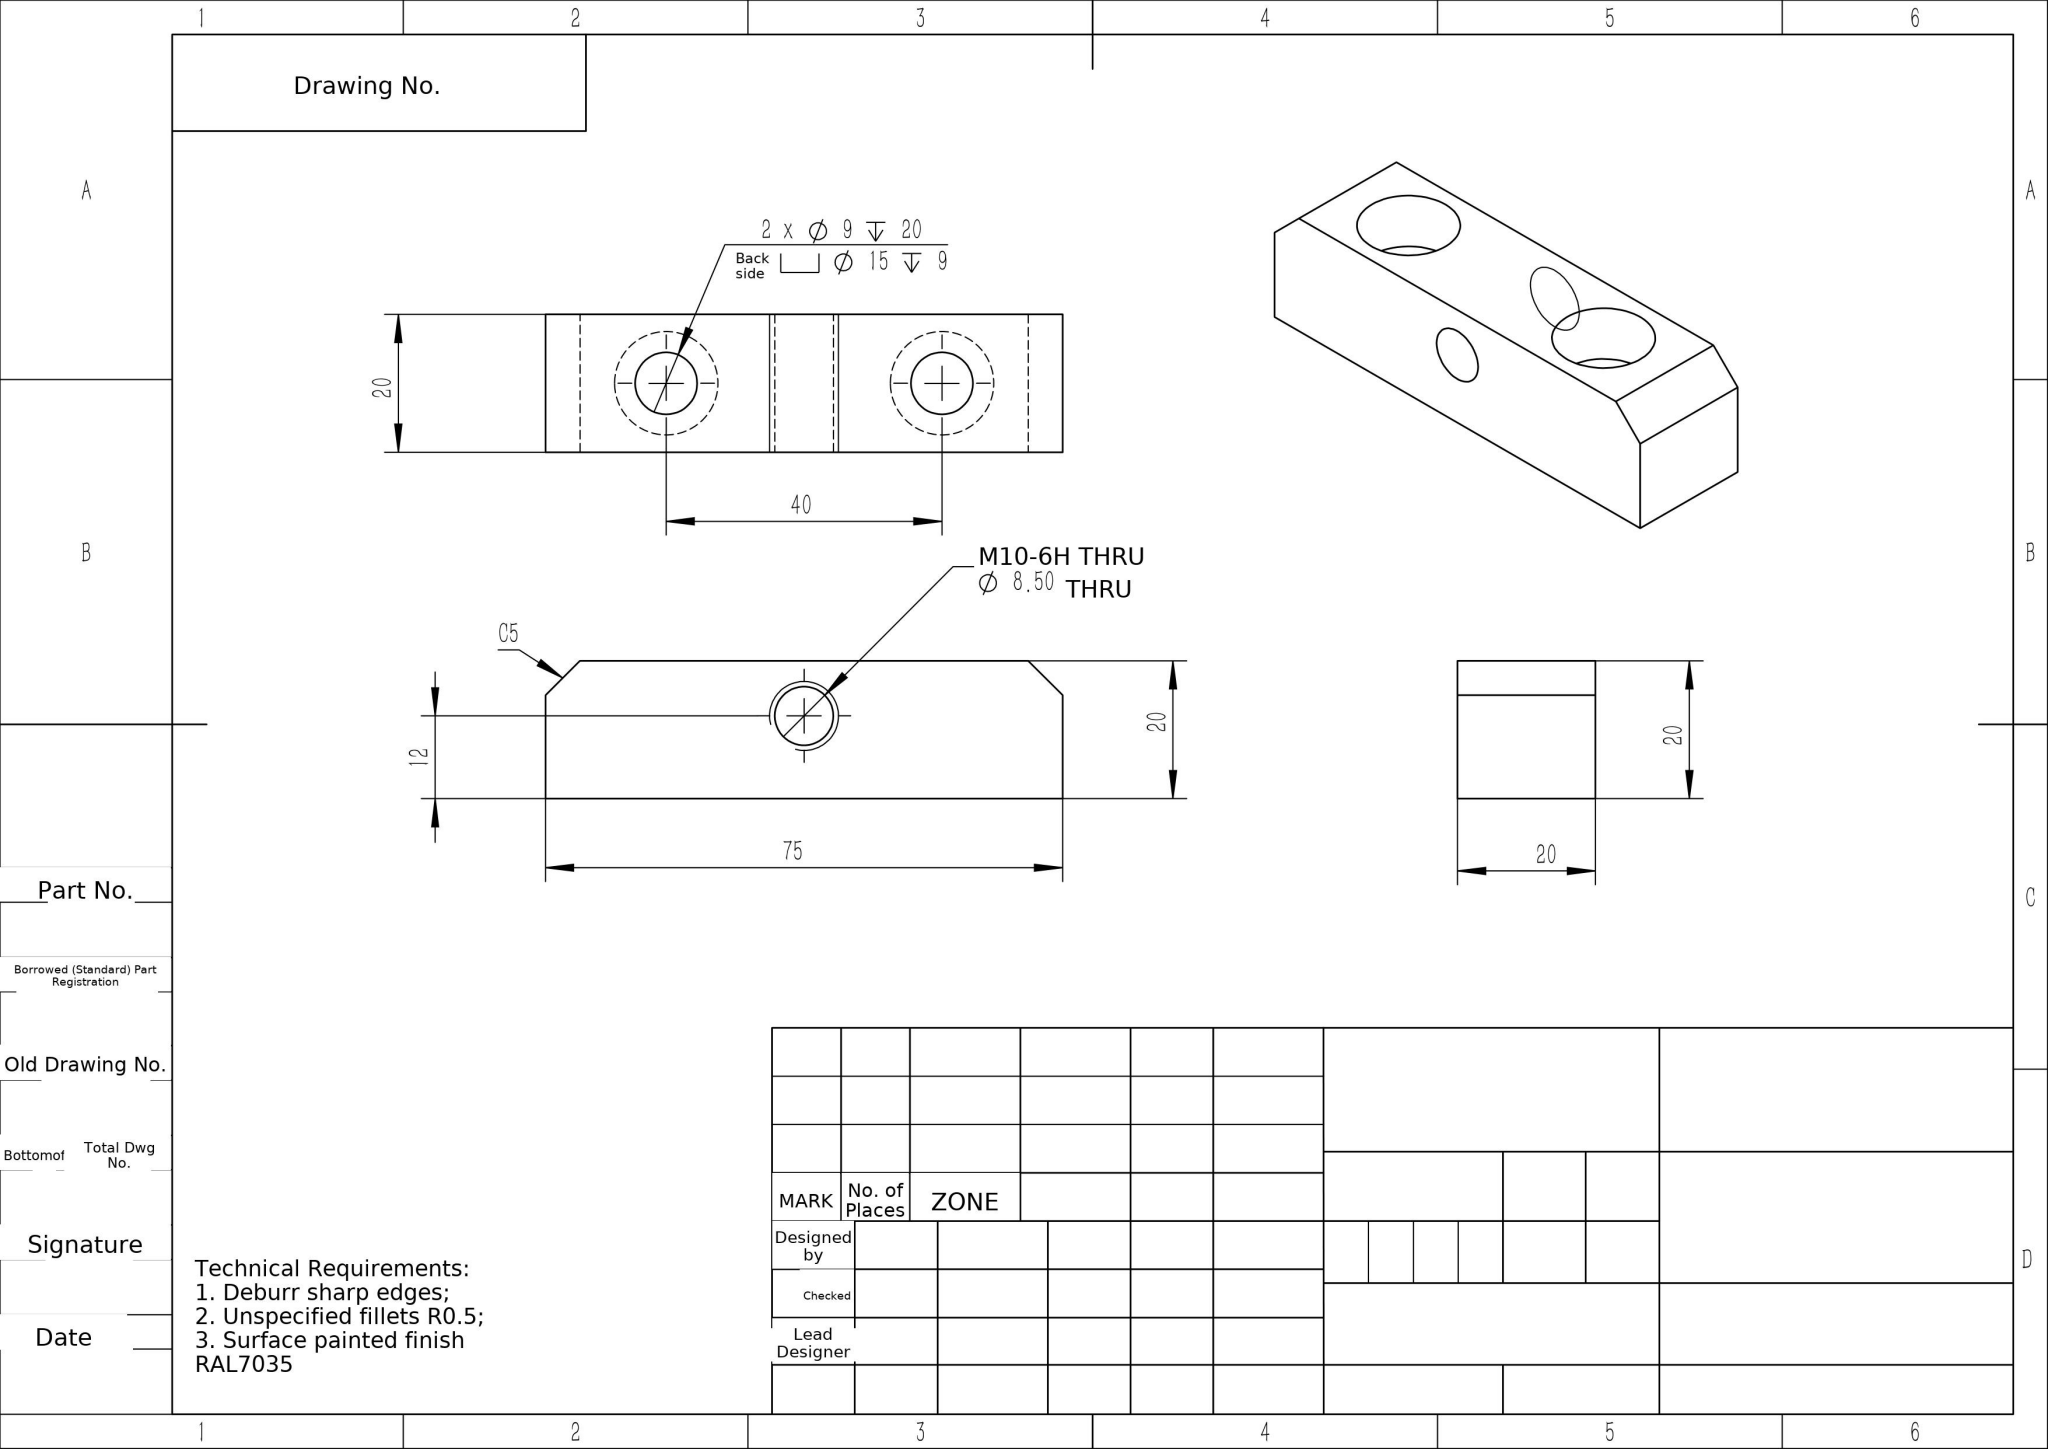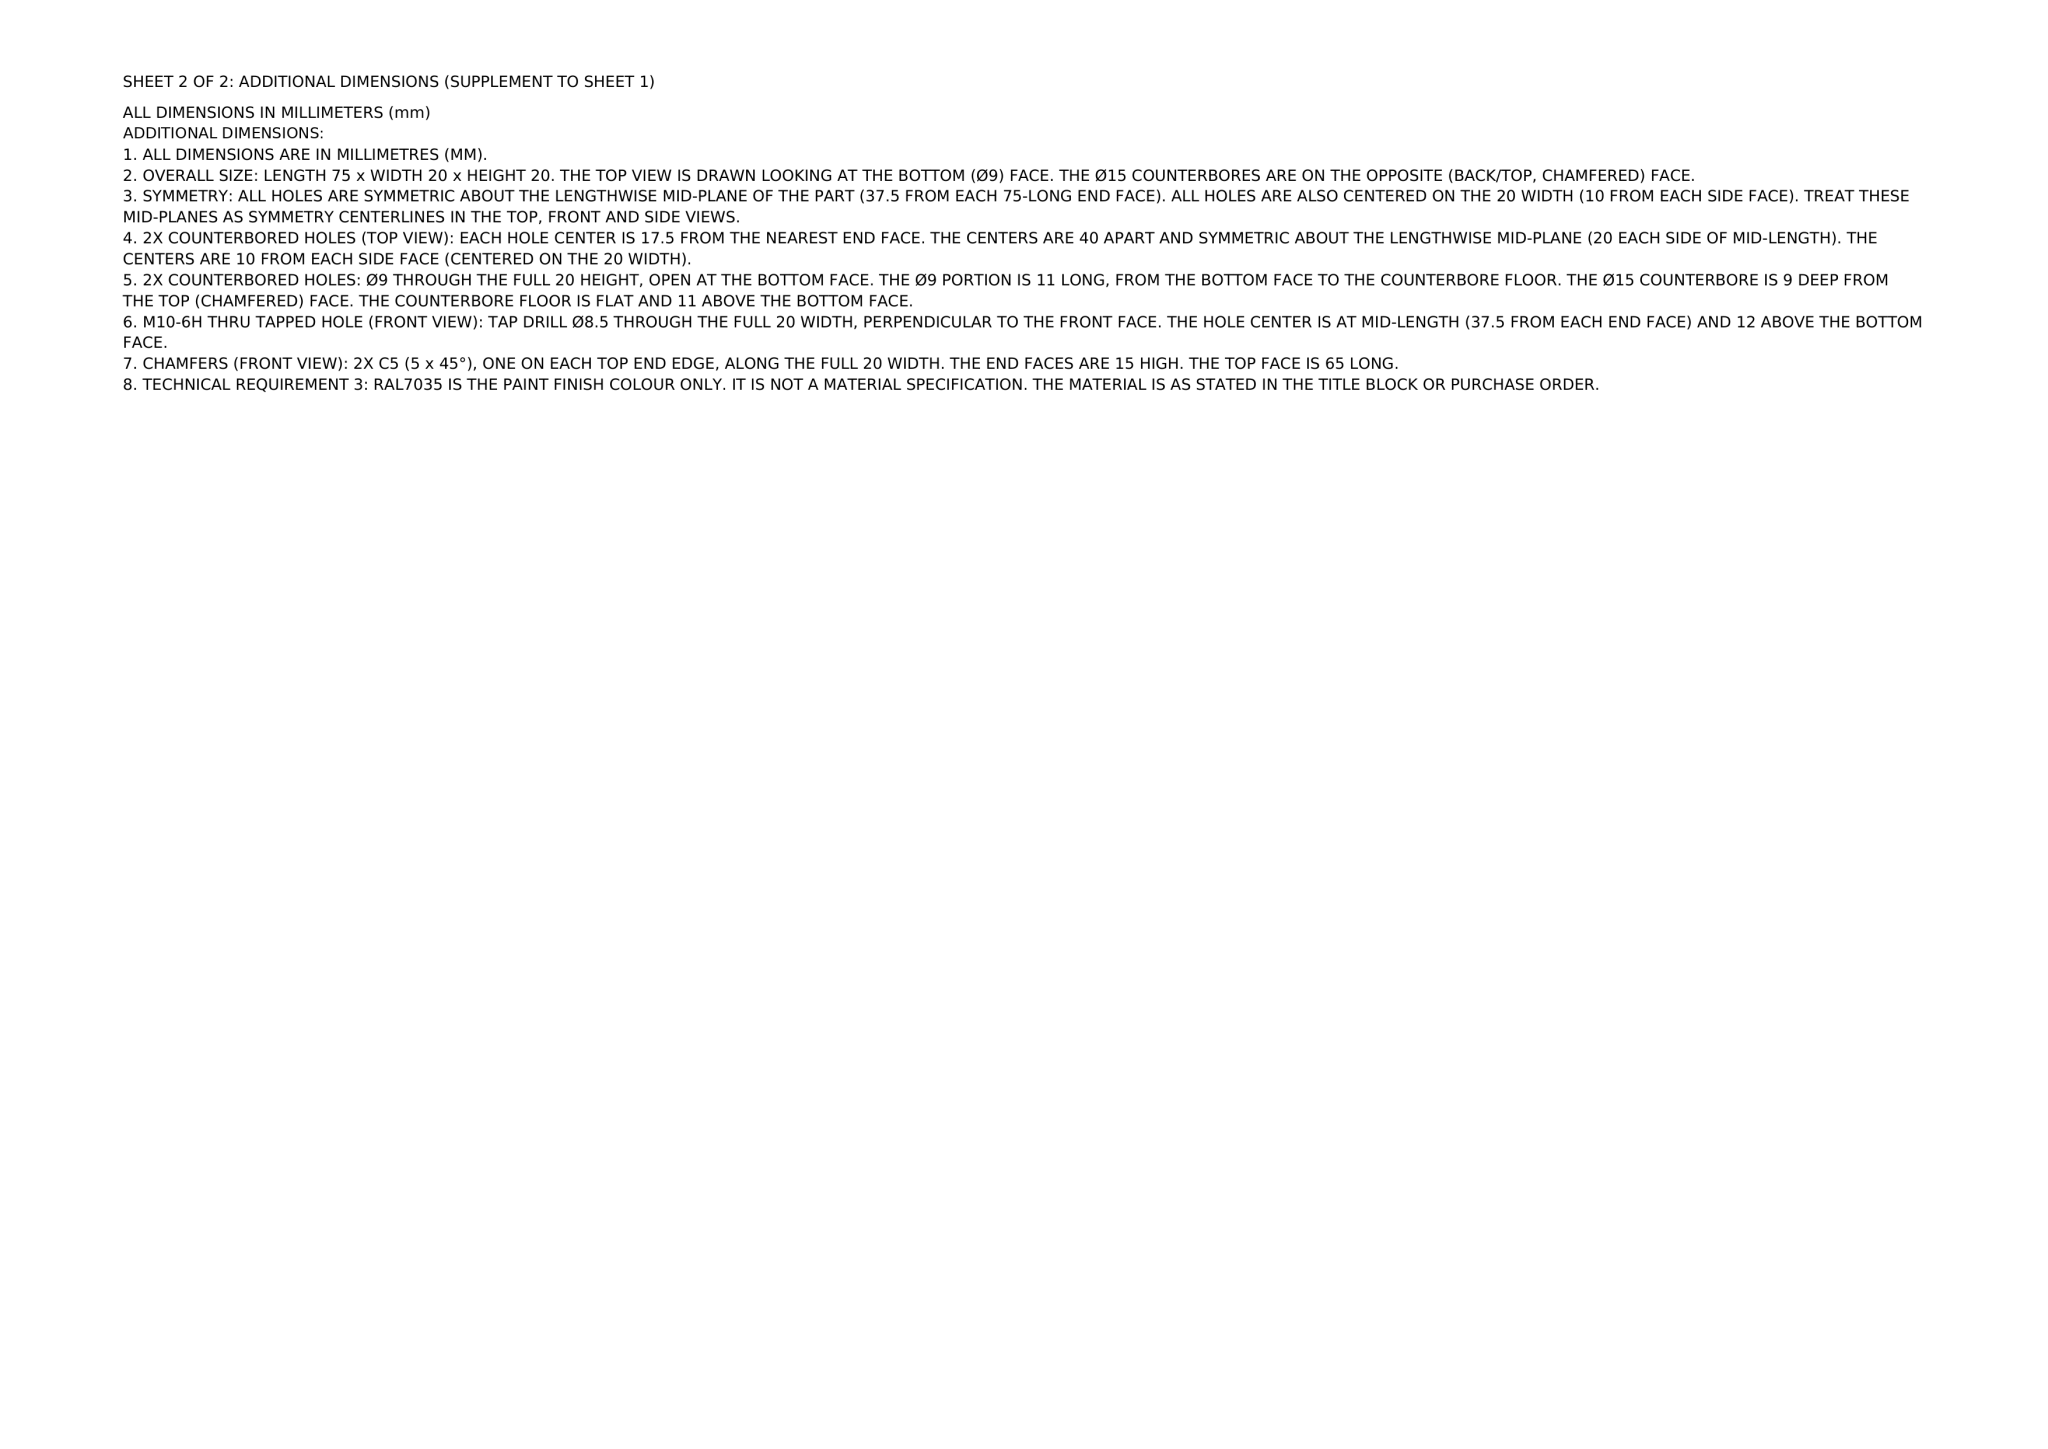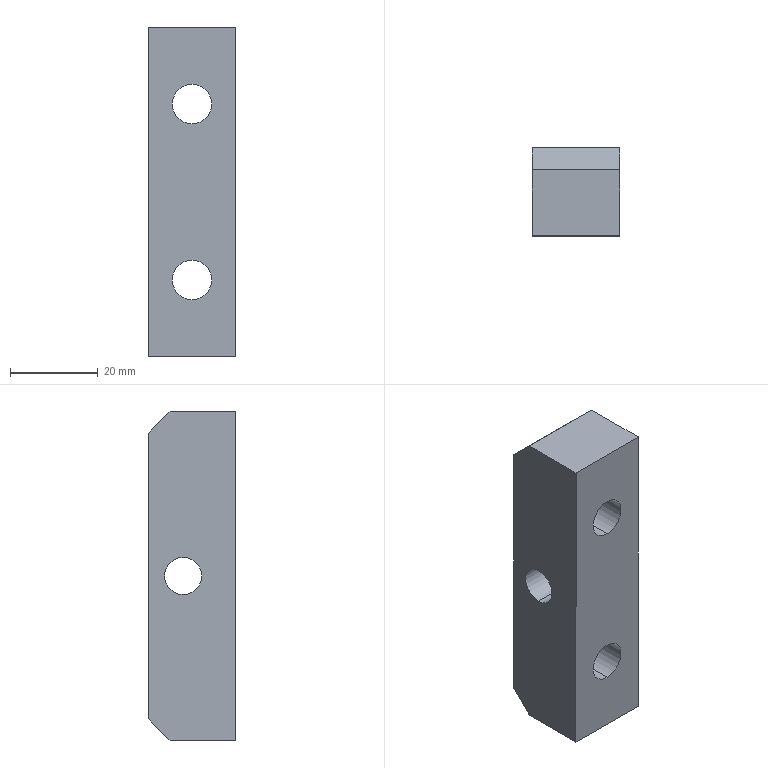Part | NX | mm | 1 solid | 20 faces | box 20 x 20 x 75 mm | volume 23785 mm3 | cylinder 10 | plane 10 | commonest cylinder face diameters 15 x4 9 x4 8.5 x2
STEP:
#1=COLOUR_RGB('',0.7765,0.7765,0.8196);
#2=FILL_AREA_STYLE_COLOUR('',#1);
#3=FILL_AREA_STYLE('',(#2));
#4=SURFACE_STYLE_FILL_AREA(#3);
#5=SURFACE_SIDE_STYLE('',(#4));
#6=SURFACE_STYLE_USAGE(.BOTH.,#5);
#7=PRESENTATION_STYLE_ASSIGNMENT((#6));
#8=CARTESIAN_POINT('',(10.,12.,-4.25));
#9=VERTEX_POINT('',#8);
#10=CARTESIAN_POINT('',(10.,12.,4.25));
#11=VERTEX_POINT('',#10);
#12=CARTESIAN_POINT('',(10.,12.,-0.));
#13=DIRECTION('',(-1.,0.,0.));
#14=DIRECTION('',(0.,0.,1.));
#15=AXIS2_PLACEMENT_3D('',#12,#13,#14);
#16=CIRCLE('',#15,4.25);
#17=EDGE_CURVE('',#9,#11,#16,.T.);
#18=ORIENTED_EDGE('',*,*,#17,.F.);
#19=CARTESIAN_POINT('',(-10.,12.,-4.25));
#20=VERTEX_POINT('',#19);
#21=CARTESIAN_POINT('',(-10.,12.,-4.25));
#22=DIRECTION('',(-1.,0.,0.));
#23=VECTOR('',#22,1000.);
#24=LINE('',#21,#23);
#25=EDGE_CURVE('',#9,#20,#24,.T.);
#26=ORIENTED_EDGE('',*,*,#25,.T.);
#27=CARTESIAN_POINT('',(-10.,12.,4.25));
#28=VERTEX_POINT('',#27);
#29=CARTESIAN_POINT('',(-10.,12.,0.));
#30=DIRECTION('',(-1.,0.,0.));
#31=DIRECTION('',(0.,0.,1.));
#32=AXIS2_PLACEMENT_3D('',#29,#30,#31);
#33=CIRCLE('',#32,4.25);
#34=EDGE_CURVE('',#20,#28,#33,.T.);
#35=ORIENTED_EDGE('',*,*,#34,.T.);
#36=CARTESIAN_POINT('',(-10.,12.,4.25));
#37=DIRECTION('',(-1.,0.,0.));
#38=VECTOR('',#37,1000.);
#39=LINE('',#36,#38);
#40=EDGE_CURVE('',#11,#28,#39,.T.);
#41=ORIENTED_EDGE('',*,*,#40,.F.);
#42=EDGE_LOOP('',(#18,#26,#35,#41));
#43=FACE_OUTER_BOUND('',#42,.T.);
#44=CARTESIAN_POINT('',(-10.,12.,0.));
#45=DIRECTION('',(-1.,0.,0.));
#46=DIRECTION('',(0.,0.,1.));
#47=AXIS2_PLACEMENT_3D('',#44,#45,#46);
#48=CYLINDRICAL_SURFACE('',#47,4.25);
#49=ADVANCED_FACE('',(#43),#48,.F.);
#50=CARTESIAN_POINT('',(0.,11.,-27.5));
#51=VERTEX_POINT('',#50);
#52=CARTESIAN_POINT('',(0.,11.,-12.5));
#53=VERTEX_POINT('',#52);
#54=CARTESIAN_POINT('',(0.,11.,-20.));
#55=DIRECTION('',(0.,1.,0.));
#56=DIRECTION('',(0.,0.,1.));
#57=AXIS2_PLACEMENT_3D('',#54,#55,#56);
#58=CIRCLE('',#57,7.5);
#59=EDGE_CURVE('',#51,#53,#58,.T.);
#60=ORIENTED_EDGE('',*,*,#59,.F.);
#61=CARTESIAN_POINT('',(0.,20.,-27.5));
#62=VERTEX_POINT('',#61);
#63=CARTESIAN_POINT('',(0.,20.,-27.5));
#64=DIRECTION('',(0.,1.,0.));
#65=VECTOR('',#64,1000.);
#66=LINE('',#63,#65);
#67=EDGE_CURVE('',#51,#62,#66,.T.);
#68=ORIENTED_EDGE('',*,*,#67,.T.);
#69=CARTESIAN_POINT('',(0.,20.,-12.5));
#70=VERTEX_POINT('',#69);
#71=CARTESIAN_POINT('',(0.,20.,-20.));
#72=DIRECTION('',(0.,1.,0.));
#73=DIRECTION('',(0.,0.,1.));
#74=AXIS2_PLACEMENT_3D('',#71,#72,#73);
#75=CIRCLE('',#74,7.5);
#76=EDGE_CURVE('',#62,#70,#75,.T.);
#77=ORIENTED_EDGE('',*,*,#76,.T.);
#78=CARTESIAN_POINT('',(0.,20.,-12.5));
#79=DIRECTION('',(0.,1.,0.));
#80=VECTOR('',#79,1000.);
#81=LINE('',#78,#80);
#82=EDGE_CURVE('',#53,#70,#81,.T.);
#83=ORIENTED_EDGE('',*,*,#82,.F.);
#84=EDGE_LOOP('',(#60,#68,#77,#83));
#85=FACE_OUTER_BOUND('',#84,.T.);
#86=CARTESIAN_POINT('',(0.,20.,-20.));
#87=DIRECTION('',(0.,1.,0.));
#88=DIRECTION('',(0.,0.,1.));
#89=AXIS2_PLACEMENT_3D('',#86,#87,#88);
#90=CYLINDRICAL_SURFACE('',#89,7.5);
#91=ADVANCED_FACE('',(#85),#90,.F.);
#92=CARTESIAN_POINT('',(0.,0.,-24.5));
#93=VERTEX_POINT('',#92);
#94=CARTESIAN_POINT('',(0.,0.,-15.5));
#95=VERTEX_POINT('',#94);
#96=CARTESIAN_POINT('',(0.,0.,-20.));
#97=DIRECTION('',(0.,1.,0.));
#98=DIRECTION('',(0.,0.,1.));
#99=AXIS2_PLACEMENT_3D('',#96,#97,#98);
#100=CIRCLE('',#99,4.5);
#101=EDGE_CURVE('',#93,#95,#100,.T.);
#102=ORIENTED_EDGE('',*,*,#101,.F.);
#103=CARTESIAN_POINT('',(0.,11.,-24.5));
#104=VERTEX_POINT('',#103);
#105=CARTESIAN_POINT('',(0.,20.,-24.5));
#106=DIRECTION('',(0.,1.,0.));
#107=VECTOR('',#106,1000.);
#108=LINE('',#105,#107);
#109=EDGE_CURVE('',#93,#104,#108,.T.);
#110=ORIENTED_EDGE('',*,*,#109,.T.);
#111=CARTESIAN_POINT('',(0.,11.,-15.5));
#112=VERTEX_POINT('',#111);
#113=CARTESIAN_POINT('',(0.,11.,-20.));
#114=DIRECTION('',(0.,1.,0.));
#115=DIRECTION('',(0.,0.,1.));
#116=AXIS2_PLACEMENT_3D('',#113,#114,#115);
#117=CIRCLE('',#116,4.5);
#118=EDGE_CURVE('',#104,#112,#117,.T.);
#119=ORIENTED_EDGE('',*,*,#118,.T.);
#120=CARTESIAN_POINT('',(0.,20.,-15.5));
#121=DIRECTION('',(0.,1.,0.));
#122=VECTOR('',#121,1000.);
#123=LINE('',#120,#122);
#124=EDGE_CURVE('',#95,#112,#123,.T.);
#125=ORIENTED_EDGE('',*,*,#124,.F.);
#126=EDGE_LOOP('',(#102,#110,#119,#125));
#127=FACE_OUTER_BOUND('',#126,.T.);
#128=CARTESIAN_POINT('',(0.,20.,-20.));
#129=DIRECTION('',(0.,1.,0.));
#130=DIRECTION('',(0.,0.,1.));
#131=AXIS2_PLACEMENT_3D('',#128,#129,#130);
#132=CYLINDRICAL_SURFACE('',#131,4.5);
#133=ADVANCED_FACE('',(#127),#132,.F.);
#134=CARTESIAN_POINT('',(0.,11.,12.5));
#135=VERTEX_POINT('',#134);
#136=CARTESIAN_POINT('',(0.,11.,27.5));
#137=VERTEX_POINT('',#136);
#138=CARTESIAN_POINT('',(0.,11.,20.));
#139=DIRECTION('',(0.,1.,0.));
#140=DIRECTION('',(0.,0.,1.));
#141=AXIS2_PLACEMENT_3D('',#138,#139,#140);
#142=CIRCLE('',#141,7.5);
#143=EDGE_CURVE('',#135,#137,#142,.T.);
#144=ORIENTED_EDGE('',*,*,#143,.F.);
#145=CARTESIAN_POINT('',(0.,20.,12.5));
#146=VERTEX_POINT('',#145);
#147=CARTESIAN_POINT('',(0.,20.,12.5));
#148=DIRECTION('',(0.,1.,0.));
#149=VECTOR('',#148,1000.);
#150=LINE('',#147,#149);
#151=EDGE_CURVE('',#135,#146,#150,.T.);
#152=ORIENTED_EDGE('',*,*,#151,.T.);
#153=CARTESIAN_POINT('',(0.,20.,27.5));
#154=VERTEX_POINT('',#153);
#155=CARTESIAN_POINT('',(0.,20.,20.));
#156=DIRECTION('',(0.,1.,0.));
#157=DIRECTION('',(0.,0.,1.));
#158=AXIS2_PLACEMENT_3D('',#155,#156,#157);
#159=CIRCLE('',#158,7.5);
#160=EDGE_CURVE('',#146,#154,#159,.T.);
#161=ORIENTED_EDGE('',*,*,#160,.T.);
#162=CARTESIAN_POINT('',(0.,20.,27.5));
#163=DIRECTION('',(0.,1.,0.));
#164=VECTOR('',#163,1000.);
#165=LINE('',#162,#164);
#166=EDGE_CURVE('',#137,#154,#165,.T.);
#167=ORIENTED_EDGE('',*,*,#166,.F.);
#168=EDGE_LOOP('',(#144,#152,#161,#167));
#169=FACE_OUTER_BOUND('',#168,.T.);
#170=CARTESIAN_POINT('',(0.,20.,20.));
#171=DIRECTION('',(0.,1.,0.));
#172=DIRECTION('',(0.,0.,1.));
#173=AXIS2_PLACEMENT_3D('',#170,#171,#172);
#174=CYLINDRICAL_SURFACE('',#173,7.5);
#175=ADVANCED_FACE('',(#169),#174,.F.);
#176=CARTESIAN_POINT('',(0.,0.,15.5));
#177=VERTEX_POINT('',#176);
#178=CARTESIAN_POINT('',(0.,0.,24.5));
#179=VERTEX_POINT('',#178);
#180=CARTESIAN_POINT('',(0.,0.,20.));
#181=DIRECTION('',(0.,1.,0.));
#182=DIRECTION('',(0.,0.,1.));
#183=AXIS2_PLACEMENT_3D('',#180,#181,#182);
#184=CIRCLE('',#183,4.5);
#185=EDGE_CURVE('',#177,#179,#184,.T.);
#186=ORIENTED_EDGE('',*,*,#185,.F.);
#187=CARTESIAN_POINT('',(0.,11.,15.5));
#188=VERTEX_POINT('',#187);
#189=CARTESIAN_POINT('',(0.,20.,15.5));
#190=DIRECTION('',(0.,1.,0.));
#191=VECTOR('',#190,1000.);
#192=LINE('',#189,#191);
#193=EDGE_CURVE('',#177,#188,#192,.T.);
#194=ORIENTED_EDGE('',*,*,#193,.T.);
#195=CARTESIAN_POINT('',(0.,11.,24.5));
#196=VERTEX_POINT('',#195);
#197=CARTESIAN_POINT('',(0.,11.,20.));
#198=DIRECTION('',(0.,1.,0.));
#199=DIRECTION('',(0.,0.,1.));
#200=AXIS2_PLACEMENT_3D('',#197,#198,#199);
#201=CIRCLE('',#200,4.5);
#202=EDGE_CURVE('',#188,#196,#201,.T.);
#203=ORIENTED_EDGE('',*,*,#202,.T.);
#204=CARTESIAN_POINT('',(0.,20.,24.5));
#205=DIRECTION('',(0.,1.,0.));
#206=VECTOR('',#205,1000.);
#207=LINE('',#204,#206);
#208=EDGE_CURVE('',#179,#196,#207,.T.);
#209=ORIENTED_EDGE('',*,*,#208,.F.);
#210=EDGE_LOOP('',(#186,#194,#203,#209));
#211=FACE_OUTER_BOUND('',#210,.T.);
#212=CARTESIAN_POINT('',(0.,20.,20.));
#213=DIRECTION('',(0.,1.,0.));
#214=DIRECTION('',(0.,0.,1.));
#215=AXIS2_PLACEMENT_3D('',#212,#213,#214);
#216=CYLINDRICAL_SURFACE('',#215,4.5);
#217=ADVANCED_FACE('',(#211),#216,.F.);
#218=CARTESIAN_POINT('',(10.,12.,-0.));
#219=DIRECTION('',(-1.,0.,0.));
#220=DIRECTION('',(0.,0.,1.));
#221=AXIS2_PLACEMENT_3D('',#218,#219,#220);
#222=CIRCLE('',#221,4.25);
#223=EDGE_CURVE('',#11,#9,#222,.T.);
#224=ORIENTED_EDGE('',*,*,#223,.T.);
#225=ORIENTED_EDGE('',*,*,#17,.T.);
#226=EDGE_LOOP('',(#224,#225));
#227=FACE_BOUND('',#226,.T.);
#228=CARTESIAN_POINT('',(10.,15.,-37.5));
#229=VERTEX_POINT('',#228);
#230=CARTESIAN_POINT('',(10.,0.,-37.5));
#231=VERTEX_POINT('',#230);
#232=CARTESIAN_POINT('',(10.,20.,-37.5));
#233=DIRECTION('',(0.,-1.,0.));
#234=VECTOR('',#233,1000.);
#235=LINE('',#232,#234);
#236=EDGE_CURVE('',#229,#231,#235,.T.);
#237=ORIENTED_EDGE('',*,*,#236,.F.);
#238=CARTESIAN_POINT('',(10.,20.,-32.5));
#239=VERTEX_POINT('',#238);
#240=CARTESIAN_POINT('',(10.,20.,-32.5));
#241=DIRECTION('',(0.,0.7071,0.7071));
#242=VECTOR('',#241,1000.);
#243=LINE('',#240,#242);
#244=EDGE_CURVE('',#229,#239,#243,.T.);
#245=ORIENTED_EDGE('',*,*,#244,.T.);
#246=CARTESIAN_POINT('',(10.,20.,32.5));
#247=VERTEX_POINT('',#246);
#248=CARTESIAN_POINT('',(10.,20.,-37.5));
#249=DIRECTION('',(-0.,0.,-1.));
#250=VECTOR('',#249,1000.);
#251=LINE('',#248,#250);
#252=EDGE_CURVE('',#247,#239,#251,.T.);
#253=ORIENTED_EDGE('',*,*,#252,.F.);
#254=CARTESIAN_POINT('',(10.,15.,37.5));
#255=VERTEX_POINT('',#254);
#256=CARTESIAN_POINT('',(10.,20.,32.5));
#257=DIRECTION('',(0.,-0.7071,0.7071));
#258=VECTOR('',#257,1000.);
#259=LINE('',#256,#258);
#260=EDGE_CURVE('',#247,#255,#259,.T.);
#261=ORIENTED_EDGE('',*,*,#260,.T.);
#262=CARTESIAN_POINT('',(10.,0.,37.5));
#263=VERTEX_POINT('',#262);
#264=CARTESIAN_POINT('',(10.,20.,37.5));
#265=DIRECTION('',(0.,-1.,0.));
#266=VECTOR('',#265,1000.);
#267=LINE('',#264,#266);
#268=EDGE_CURVE('',#255,#263,#267,.T.);
#269=ORIENTED_EDGE('',*,*,#268,.T.);
#270=CARTESIAN_POINT('',(10.,0.,-37.5));
#271=DIRECTION('',(-0.,0.,-1.));
#272=VECTOR('',#271,1000.);
#273=LINE('',#270,#272);
#274=EDGE_CURVE('',#263,#231,#273,.T.);
#275=ORIENTED_EDGE('',*,*,#274,.T.);
#276=EDGE_LOOP('',(#237,#245,#253,#261,#269,#275));
#277=FACE_OUTER_BOUND('',#276,.T.);
#278=CARTESIAN_POINT('',(10.,20.,-37.5));
#279=DIRECTION('',(-1.,0.,0.));
#280=DIRECTION('',(0.,0.,1.));
#281=AXIS2_PLACEMENT_3D('',#278,#279,#280);
#282=PLANE('',#281);
#283=ADVANCED_FACE('',(#227,#277),#282,.F.);
#284=CARTESIAN_POINT('',(-10.,15.,-37.5));
#285=VERTEX_POINT('',#284);
#286=CARTESIAN_POINT('',(-10.,0.,-37.5));
#287=VERTEX_POINT('',#286);
#288=CARTESIAN_POINT('',(-10.,20.,-37.5));
#289=DIRECTION('',(0.,-1.,0.));
#290=VECTOR('',#289,1000.);
#291=LINE('',#288,#290);
#292=EDGE_CURVE('',#285,#287,#291,.T.);
#293=ORIENTED_EDGE('',*,*,#292,.F.);
#294=CARTESIAN_POINT('',(10.,15.,-37.5));
#295=DIRECTION('',(1.,0.,0.));
#296=VECTOR('',#295,1000.);
#297=LINE('',#294,#296);
#298=EDGE_CURVE('',#285,#229,#297,.T.);
#299=ORIENTED_EDGE('',*,*,#298,.T.);
#300=ORIENTED_EDGE('',*,*,#236,.T.);
#301=CARTESIAN_POINT('',(-10.,0.,-37.5));
#302=DIRECTION('',(-1.,0.,0.));
#303=VECTOR('',#302,1000.);
#304=LINE('',#301,#303);
#305=EDGE_CURVE('',#231,#287,#304,.T.);
#306=ORIENTED_EDGE('',*,*,#305,.T.);
#307=EDGE_LOOP('',(#293,#299,#300,#306));
#308=FACE_OUTER_BOUND('',#307,.T.);
#309=CARTESIAN_POINT('',(-10.,20.,-37.5));
#310=DIRECTION('',(0.,0.,1.));
#311=DIRECTION('',(1.,0.,0.));
#312=AXIS2_PLACEMENT_3D('',#309,#310,#311);
#313=PLANE('',#312);
#314=ADVANCED_FACE('',(#308),#313,.F.);
#315=CARTESIAN_POINT('',(-10.,12.,0.));
#316=DIRECTION('',(-1.,0.,0.));
#317=DIRECTION('',(0.,0.,1.));
#318=AXIS2_PLACEMENT_3D('',#315,#316,#317);
#319=CIRCLE('',#318,4.25);
#320=EDGE_CURVE('',#28,#20,#319,.T.);
#321=ORIENTED_EDGE('',*,*,#320,.F.);
#322=ORIENTED_EDGE('',*,*,#34,.F.);
#323=EDGE_LOOP('',(#321,#322));
#324=FACE_BOUND('',#323,.T.);
#325=CARTESIAN_POINT('',(-10.,20.,-32.5));
#326=VERTEX_POINT('',#325);
#327=CARTESIAN_POINT('',(-10.,20.,32.5));
#328=VERTEX_POINT('',#327);
#329=CARTESIAN_POINT('',(-10.,20.,-37.5));
#330=DIRECTION('',(0.,0.,1.));
#331=VECTOR('',#330,1000.);
#332=LINE('',#329,#331);
#333=EDGE_CURVE('',#326,#328,#332,.T.);
#334=ORIENTED_EDGE('',*,*,#333,.F.);
#335=CARTESIAN_POINT('',(-10.,20.,-32.5));
#336=DIRECTION('',(-0.,-0.7071,-0.7071));
#337=VECTOR('',#336,1000.);
#338=LINE('',#335,#337);
#339=EDGE_CURVE('',#326,#285,#338,.T.);
#340=ORIENTED_EDGE('',*,*,#339,.T.);
#341=ORIENTED_EDGE('',*,*,#292,.T.);
#342=CARTESIAN_POINT('',(-10.,0.,37.5));
#343=VERTEX_POINT('',#342);
#344=CARTESIAN_POINT('',(-10.,0.,-37.5));
#345=DIRECTION('',(0.,0.,1.));
#346=VECTOR('',#345,1000.);
#347=LINE('',#344,#346);
#348=EDGE_CURVE('',#287,#343,#347,.T.);
#349=ORIENTED_EDGE('',*,*,#348,.T.);
#350=CARTESIAN_POINT('',(-10.,15.,37.5));
#351=VERTEX_POINT('',#350);
#352=CARTESIAN_POINT('',(-10.,20.,37.5));
#353=DIRECTION('',(0.,-1.,0.));
#354=VECTOR('',#353,1000.);
#355=LINE('',#352,#354);
#356=EDGE_CURVE('',#351,#343,#355,.T.);
#357=ORIENTED_EDGE('',*,*,#356,.F.);
#358=CARTESIAN_POINT('',(-10.,20.,32.5));
#359=DIRECTION('',(-0.,0.7071,-0.7071));
#360=VECTOR('',#359,1000.);
#361=LINE('',#358,#360);
#362=EDGE_CURVE('',#351,#328,#361,.T.);
#363=ORIENTED_EDGE('',*,*,#362,.T.);
#364=EDGE_LOOP('',(#334,#340,#341,#349,#357,#363));
#365=FACE_OUTER_BOUND('',#364,.T.);
#366=CARTESIAN_POINT('',(-10.,20.,-37.5));
#367=DIRECTION('',(1.,0.,-0.));
#368=DIRECTION('',(-0.,0.,-1.));
#369=AXIS2_PLACEMENT_3D('',#366,#367,#368);
#370=PLANE('',#369);
#371=ADVANCED_FACE('',(#324,#365),#370,.F.);
#372=ORIENTED_EDGE('',*,*,#268,.F.);
#373=CARTESIAN_POINT('',(-10.,15.,37.5));
#374=DIRECTION('',(-1.,0.,0.));
#375=VECTOR('',#374,1000.);
#376=LINE('',#373,#375);
#377=EDGE_CURVE('',#255,#351,#376,.T.);
#378=ORIENTED_EDGE('',*,*,#377,.T.);
#379=ORIENTED_EDGE('',*,*,#356,.T.);
#380=CARTESIAN_POINT('',(-10.,0.,37.5));
#381=DIRECTION('',(1.,0.,0.));
#382=VECTOR('',#381,1000.);
#383=LINE('',#380,#382);
#384=EDGE_CURVE('',#343,#263,#383,.T.);
#385=ORIENTED_EDGE('',*,*,#384,.T.);
#386=EDGE_LOOP('',(#372,#378,#379,#385));
#387=FACE_OUTER_BOUND('',#386,.T.);
#388=CARTESIAN_POINT('',(-10.,20.,37.5));
#389=DIRECTION('',(0.,0.,-1.));
#390=DIRECTION('',(-1.,0.,0.));
#391=AXIS2_PLACEMENT_3D('',#388,#389,#390);
#392=PLANE('',#391);
#393=ADVANCED_FACE('',(#387),#392,.F.);
#394=CARTESIAN_POINT('',(0.,20.,-20.));
#395=DIRECTION('',(0.,1.,0.));
#396=DIRECTION('',(0.,0.,1.));
#397=AXIS2_PLACEMENT_3D('',#394,#395,#396);
#398=CIRCLE('',#397,7.5);
#399=EDGE_CURVE('',#70,#62,#398,.T.);
#400=ORIENTED_EDGE('',*,*,#399,.F.);
#401=ORIENTED_EDGE('',*,*,#76,.F.);
#402=EDGE_LOOP('',(#400,#401));
#403=FACE_BOUND('',#402,.T.);
#404=CARTESIAN_POINT('',(0.,20.,20.));
#405=DIRECTION('',(0.,1.,0.));
#406=DIRECTION('',(0.,0.,1.));
#407=AXIS2_PLACEMENT_3D('',#404,#405,#406);
#408=CIRCLE('',#407,7.5);
#409=EDGE_CURVE('',#154,#146,#408,.T.);
#410=ORIENTED_EDGE('',*,*,#409,.F.);
#411=ORIENTED_EDGE('',*,*,#160,.F.);
#412=EDGE_LOOP('',(#410,#411));
#413=FACE_BOUND('',#412,.T.);
#414=ORIENTED_EDGE('',*,*,#252,.T.);
#415=CARTESIAN_POINT('',(-10.,20.,-32.5));
#416=DIRECTION('',(-1.,0.,0.));
#417=VECTOR('',#416,1000.);
#418=LINE('',#415,#417);
#419=EDGE_CURVE('',#239,#326,#418,.T.);
#420=ORIENTED_EDGE('',*,*,#419,.T.);
#421=ORIENTED_EDGE('',*,*,#333,.T.);
#422=CARTESIAN_POINT('',(10.,20.,32.5));
#423=DIRECTION('',(1.,0.,0.));
#424=VECTOR('',#423,1000.);
#425=LINE('',#422,#424);
#426=EDGE_CURVE('',#328,#247,#425,.T.);
#427=ORIENTED_EDGE('',*,*,#426,.T.);
#428=EDGE_LOOP('',(#414,#420,#421,#427));
#429=FACE_OUTER_BOUND('',#428,.T.);
#430=CARTESIAN_POINT('',(0.,20.,0.));
#431=DIRECTION('',(0.,1.,0.));
#432=DIRECTION('',(0.,0.,1.));
#433=AXIS2_PLACEMENT_3D('',#430,#431,#432);
#434=PLANE('',#433);
#435=ADVANCED_FACE('',(#403,#413,#429),#434,.T.);
#436=CARTESIAN_POINT('',(0.,0.,-20.));
#437=DIRECTION('',(0.,1.,0.));
#438=DIRECTION('',(0.,0.,1.));
#439=AXIS2_PLACEMENT_3D('',#436,#437,#438);
#440=CIRCLE('',#439,4.5);
#441=EDGE_CURVE('',#95,#93,#440,.T.);
#442=ORIENTED_EDGE('',*,*,#441,.T.);
#443=ORIENTED_EDGE('',*,*,#101,.T.);
#444=EDGE_LOOP('',(#442,#443));
#445=FACE_BOUND('',#444,.T.);
#446=CARTESIAN_POINT('',(0.,0.,20.));
#447=DIRECTION('',(0.,1.,0.));
#448=DIRECTION('',(0.,0.,1.));
#449=AXIS2_PLACEMENT_3D('',#446,#447,#448);
#450=CIRCLE('',#449,4.5);
#451=EDGE_CURVE('',#179,#177,#450,.T.);
#452=ORIENTED_EDGE('',*,*,#451,.T.);
#453=ORIENTED_EDGE('',*,*,#185,.T.);
#454=EDGE_LOOP('',(#452,#453));
#455=FACE_BOUND('',#454,.T.);
#456=ORIENTED_EDGE('',*,*,#274,.F.);
#457=ORIENTED_EDGE('',*,*,#384,.F.);
#458=ORIENTED_EDGE('',*,*,#348,.F.);
#459=ORIENTED_EDGE('',*,*,#305,.F.);
#460=EDGE_LOOP('',(#456,#457,#458,#459));
#461=FACE_OUTER_BOUND('',#460,.T.);
#462=CARTESIAN_POINT('',(0.,0.,0.));
#463=DIRECTION('',(0.,1.,0.));
#464=DIRECTION('',(0.,0.,1.));
#465=AXIS2_PLACEMENT_3D('',#462,#463,#464);
#466=PLANE('',#465);
#467=ADVANCED_FACE('',(#445,#455,#461),#466,.F.);
#468=ORIENTED_EDGE('',*,*,#244,.F.);
#469=ORIENTED_EDGE('',*,*,#298,.F.);
#470=ORIENTED_EDGE('',*,*,#339,.F.);
#471=ORIENTED_EDGE('',*,*,#419,.F.);
#472=EDGE_LOOP('',(#468,#469,#470,#471));
#473=FACE_OUTER_BOUND('',#472,.T.);
#474=CARTESIAN_POINT('',(0.,20.,-32.5));
#475=DIRECTION('',(0.,0.7071,-0.7071));
#476=DIRECTION('',(1.,0.,0.));
#477=AXIS2_PLACEMENT_3D('',#474,#475,#476);
#478=PLANE('',#477);
#479=ADVANCED_FACE('',(#473),#478,.T.);
#480=ORIENTED_EDGE('',*,*,#362,.F.);
#481=ORIENTED_EDGE('',*,*,#377,.F.);
#482=ORIENTED_EDGE('',*,*,#260,.F.);
#483=ORIENTED_EDGE('',*,*,#426,.F.);
#484=EDGE_LOOP('',(#480,#481,#482,#483));
#485=FACE_OUTER_BOUND('',#484,.T.);
#486=CARTESIAN_POINT('',(0.,20.,32.5));
#487=DIRECTION('',(0.,0.7071,0.7071));
#488=DIRECTION('',(-1.,0.,0.));
#489=AXIS2_PLACEMENT_3D('',#486,#487,#488);
#490=PLANE('',#489);
#491=ADVANCED_FACE('',(#485),#490,.T.);
#492=ORIENTED_EDGE('',*,*,#193,.F.);
#493=ORIENTED_EDGE('',*,*,#451,.F.);
#494=ORIENTED_EDGE('',*,*,#208,.T.);
#495=CARTESIAN_POINT('',(0.,11.,20.));
#496=DIRECTION('',(0.,1.,0.));
#497=DIRECTION('',(0.,0.,1.));
#498=AXIS2_PLACEMENT_3D('',#495,#496,#497);
#499=CIRCLE('',#498,4.5);
#500=EDGE_CURVE('',#196,#188,#499,.T.);
#501=ORIENTED_EDGE('',*,*,#500,.T.);
#502=EDGE_LOOP('',(#492,#493,#494,#501));
#503=FACE_OUTER_BOUND('',#502,.T.);
#504=CARTESIAN_POINT('',(0.,20.,20.));
#505=DIRECTION('',(0.,1.,0.));
#506=DIRECTION('',(0.,0.,1.));
#507=AXIS2_PLACEMENT_3D('',#504,#505,#506);
#508=CYLINDRICAL_SURFACE('',#507,4.5);
#509=ADVANCED_FACE('',(#503),#508,.F.);
#510=ORIENTED_EDGE('',*,*,#500,.F.);
#511=ORIENTED_EDGE('',*,*,#202,.F.);
#512=EDGE_LOOP('',(#510,#511));
#513=FACE_BOUND('',#512,.T.);
#514=CARTESIAN_POINT('',(0.,11.,20.));
#515=DIRECTION('',(0.,1.,0.));
#516=DIRECTION('',(0.,0.,1.));
#517=AXIS2_PLACEMENT_3D('',#514,#515,#516);
#518=CIRCLE('',#517,7.5);
#519=EDGE_CURVE('',#137,#135,#518,.T.);
#520=ORIENTED_EDGE('',*,*,#519,.T.);
#521=ORIENTED_EDGE('',*,*,#143,.T.);
#522=EDGE_LOOP('',(#520,#521));
#523=FACE_OUTER_BOUND('',#522,.T.);
#524=CARTESIAN_POINT('',(4.5,11.,20.));
#525=DIRECTION('',(0.,-1.,0.));
#526=DIRECTION('',(0.,0.,-1.));
#527=AXIS2_PLACEMENT_3D('',#524,#525,#526);
#528=PLANE('',#527);
#529=ADVANCED_FACE('',(#513,#523),#528,.F.);
#530=ORIENTED_EDGE('',*,*,#151,.F.);
#531=ORIENTED_EDGE('',*,*,#519,.F.);
#532=ORIENTED_EDGE('',*,*,#166,.T.);
#533=ORIENTED_EDGE('',*,*,#409,.T.);
#534=EDGE_LOOP('',(#530,#531,#532,#533));
#535=FACE_OUTER_BOUND('',#534,.T.);
#536=CARTESIAN_POINT('',(0.,20.,20.));
#537=DIRECTION('',(0.,1.,0.));
#538=DIRECTION('',(0.,0.,1.));
#539=AXIS2_PLACEMENT_3D('',#536,#537,#538);
#540=CYLINDRICAL_SURFACE('',#539,7.5);
#541=ADVANCED_FACE('',(#535),#540,.F.);
#542=ORIENTED_EDGE('',*,*,#109,.F.);
#543=ORIENTED_EDGE('',*,*,#441,.F.);
#544=ORIENTED_EDGE('',*,*,#124,.T.);
#545=CARTESIAN_POINT('',(0.,11.,-20.));
#546=DIRECTION('',(0.,1.,0.));
#547=DIRECTION('',(0.,0.,1.));
#548=AXIS2_PLACEMENT_3D('',#545,#546,#547);
#549=CIRCLE('',#548,4.5);
#550=EDGE_CURVE('',#112,#104,#549,.T.);
#551=ORIENTED_EDGE('',*,*,#550,.T.);
#552=EDGE_LOOP('',(#542,#543,#544,#551));
#553=FACE_OUTER_BOUND('',#552,.T.);
#554=CARTESIAN_POINT('',(0.,20.,-20.));
#555=DIRECTION('',(0.,1.,0.));
#556=DIRECTION('',(0.,0.,1.));
#557=AXIS2_PLACEMENT_3D('',#554,#555,#556);
#558=CYLINDRICAL_SURFACE('',#557,4.5);
#559=ADVANCED_FACE('',(#553),#558,.F.);
#560=ORIENTED_EDGE('',*,*,#550,.F.);
#561=ORIENTED_EDGE('',*,*,#118,.F.);
#562=EDGE_LOOP('',(#560,#561));
#563=FACE_BOUND('',#562,.T.);
#564=CARTESIAN_POINT('',(0.,11.,-20.));
#565=DIRECTION('',(0.,1.,0.));
#566=DIRECTION('',(0.,0.,1.));
#567=AXIS2_PLACEMENT_3D('',#564,#565,#566);
#568=CIRCLE('',#567,7.5);
#569=EDGE_CURVE('',#53,#51,#568,.T.);
#570=ORIENTED_EDGE('',*,*,#569,.T.);
#571=ORIENTED_EDGE('',*,*,#59,.T.);
#572=EDGE_LOOP('',(#570,#571));
#573=FACE_OUTER_BOUND('',#572,.T.);
#574=CARTESIAN_POINT('',(4.5,11.,-20.));
#575=DIRECTION('',(0.,-1.,0.));
#576=DIRECTION('',(0.,0.,-1.));
#577=AXIS2_PLACEMENT_3D('',#574,#575,#576);
#578=PLANE('',#577);
#579=ADVANCED_FACE('',(#563,#573),#578,.F.);
#580=ORIENTED_EDGE('',*,*,#67,.F.);
#581=ORIENTED_EDGE('',*,*,#569,.F.);
#582=ORIENTED_EDGE('',*,*,#82,.T.);
#583=ORIENTED_EDGE('',*,*,#399,.T.);
#584=EDGE_LOOP('',(#580,#581,#582,#583));
#585=FACE_OUTER_BOUND('',#584,.T.);
#586=CARTESIAN_POINT('',(0.,20.,-20.));
#587=DIRECTION('',(0.,1.,0.));
#588=DIRECTION('',(0.,0.,1.));
#589=AXIS2_PLACEMENT_3D('',#586,#587,#588);
#590=CYLINDRICAL_SURFACE('',#589,7.5);
#591=ADVANCED_FACE('',(#585),#590,.F.);
#592=ORIENTED_EDGE('',*,*,#25,.F.);
#593=ORIENTED_EDGE('',*,*,#223,.F.);
#594=ORIENTED_EDGE('',*,*,#40,.T.);
#595=ORIENTED_EDGE('',*,*,#320,.T.);
#596=EDGE_LOOP('',(#592,#593,#594,#595));
#597=FACE_OUTER_BOUND('',#596,.T.);
#598=CARTESIAN_POINT('',(-10.,12.,0.));
#599=DIRECTION('',(-1.,0.,0.));
#600=DIRECTION('',(0.,0.,1.));
#601=AXIS2_PLACEMENT_3D('',#598,#599,#600);
#602=CYLINDRICAL_SURFACE('',#601,4.25);
#603=ADVANCED_FACE('',(#597),#602,.F.);
#604=CLOSED_SHELL('',(#49,#91,#133,#175,#217,#283,#314,#371,#393,#435,#467,#479,#491,#509,#529,#541,#559,#579,#591,#603));
#605=MANIFOLD_SOLID_BREP('',#604);
#606=CARTESIAN_POINT('',(0.,0.,0.));
#607=DIRECTION('',(0.,0.,1.));
#608=DIRECTION('',(1.,0.,0.));
#609=AXIS2_PLACEMENT_3D('',#606,#607,#608);
#610=(LENGTH_UNIT()NAMED_UNIT(*)SI_UNIT(.MILLI.,.METRE.));
#611=UNCERTAINTY_MEASURE_WITH_UNIT(LENGTH_MEASURE(0.00001),#610,'','');
#612=(NAMED_UNIT(*)PLANE_ANGLE_UNIT()SI_UNIT($,.RADIAN.));
#613=(NAMED_UNIT(*)SI_UNIT($,.STERADIAN.)SOLID_ANGLE_UNIT());
#614=(GEOMETRIC_REPRESENTATION_CONTEXT(3)GLOBAL_UNCERTAINTY_ASSIGNED_CONTEXT((#611))GLOBAL_UNIT_ASSIGNED_CONTEXT((#610,#612,#613))REPRESENTATION_CONTEXT('',''));
#615=ADVANCED_BREP_SHAPE_REPRESENTATION('',(#605,#609),#614);
#616=STYLED_ITEM('',(#7),#615);
#617=(LENGTH_UNIT()NAMED_UNIT(*)SI_UNIT(.MILLI.,.METRE.));
#618=UNCERTAINTY_MEASURE_WITH_UNIT(LENGTH_MEASURE(0.00001),#617,'','');
#619=(NAMED_UNIT(*)PLANE_ANGLE_UNIT()SI_UNIT($,.RADIAN.));
#620=(NAMED_UNIT(*)SI_UNIT($,.STERADIAN.)SOLID_ANGLE_UNIT());
#621=(GEOMETRIC_REPRESENTATION_CONTEXT(3)GLOBAL_UNCERTAINTY_ASSIGNED_CONTEXT((#618))GLOBAL_UNIT_ASSIGNED_CONTEXT((#617,#619,#620))REPRESENTATION_CONTEXT('',''));
#622=MECHANICAL_DESIGN_GEOMETRIC_PRESENTATION_REPRESENTATION('',(#616),#621);
#623=COLOUR_RGB('',1.,1.,1.);
#624=FILL_AREA_STYLE_COLOUR('',#623);
#625=FILL_AREA_STYLE('',(#624));
#626=SURFACE_STYLE_FILL_AREA(#625);
#627=SURFACE_SIDE_STYLE('',(#626));
#628=SURFACE_STYLE_USAGE(.BOTH.,#627);
#629=PRESENTATION_STYLE_ASSIGNMENT((#628));
#630=STYLED_ITEM('',(#629),#49);
#631=(LENGTH_UNIT()NAMED_UNIT(*)SI_UNIT(.MILLI.,.METRE.));
#632=UNCERTAINTY_MEASURE_WITH_UNIT(LENGTH_MEASURE(0.00001),#631,'','');
#633=(NAMED_UNIT(*)PLANE_ANGLE_UNIT()SI_UNIT($,.RADIAN.));
#634=(NAMED_UNIT(*)SI_UNIT($,.STERADIAN.)SOLID_ANGLE_UNIT());
#635=(GEOMETRIC_REPRESENTATION_CONTEXT(3)GLOBAL_UNCERTAINTY_ASSIGNED_CONTEXT((#632))GLOBAL_UNIT_ASSIGNED_CONTEXT((#631,#633,#634))REPRESENTATION_CONTEXT('',''));
#636=MECHANICAL_DESIGN_GEOMETRIC_PRESENTATION_REPRESENTATION('',(#630),#635);
#637=COLOUR_RGB('',1.,1.,1.);
#638=FILL_AREA_STYLE_COLOUR('',#637);
#639=FILL_AREA_STYLE('',(#638));
#640=SURFACE_STYLE_FILL_AREA(#639);
#641=SURFACE_SIDE_STYLE('',(#640));
#642=SURFACE_STYLE_USAGE(.BOTH.,#641);
#643=PRESENTATION_STYLE_ASSIGNMENT((#642));
#644=STYLED_ITEM('',(#643),#603);
#645=(LENGTH_UNIT()NAMED_UNIT(*)SI_UNIT(.MILLI.,.METRE.));
#646=UNCERTAINTY_MEASURE_WITH_UNIT(LENGTH_MEASURE(0.00001),#645,'','');
#647=(NAMED_UNIT(*)PLANE_ANGLE_UNIT()SI_UNIT($,.RADIAN.));
#648=(NAMED_UNIT(*)SI_UNIT($,.STERADIAN.)SOLID_ANGLE_UNIT());
#649=(GEOMETRIC_REPRESENTATION_CONTEXT(3)GLOBAL_UNCERTAINTY_ASSIGNED_CONTEXT((#646))GLOBAL_UNIT_ASSIGNED_CONTEXT((#645,#647,#648))REPRESENTATION_CONTEXT('',''));
#650=MECHANICAL_DESIGN_GEOMETRIC_PRESENTATION_REPRESENTATION('',(#644),#649);
#651=PRESENTATION_LAYER_ASSIGNMENT('','',(#616));
#652=COLOUR_RGB('',0.7765,0.7765,0.8196);
#653=FILL_AREA_STYLE_COLOUR('',#652);
#654=FILL_AREA_STYLE('',(#653));
#655=SURFACE_STYLE_FILL_AREA(#654);
#656=SURFACE_SIDE_STYLE('',(#655));
#657=SURFACE_STYLE_USAGE(.BOTH.,#656);
#658=PRESENTATION_STYLE_ASSIGNMENT((#657));
#659=STYLED_ITEM('',(#658),#605);
#660=(LENGTH_UNIT()NAMED_UNIT(*)SI_UNIT(.MILLI.,.METRE.));
#661=UNCERTAINTY_MEASURE_WITH_UNIT(LENGTH_MEASURE(0.00001),#660,'','');
#662=(NAMED_UNIT(*)PLANE_ANGLE_UNIT()SI_UNIT($,.RADIAN.));
#663=(NAMED_UNIT(*)SI_UNIT($,.STERADIAN.)SOLID_ANGLE_UNIT());
#664=(GEOMETRIC_REPRESENTATION_CONTEXT(3)GLOBAL_UNCERTAINTY_ASSIGNED_CONTEXT((#661))GLOBAL_UNIT_ASSIGNED_CONTEXT((#660,#662,#663))REPRESENTATION_CONTEXT('',''));
#665=MECHANICAL_DESIGN_GEOMETRIC_PRESENTATION_REPRESENTATION('',(#659),#664);
#666=PRESENTATION_LAYER_ASSIGNMENT('','',(#630));
#667=PRESENTATION_LAYER_ASSIGNMENT('','',(#659));
#668=PRESENTATION_LAYER_ASSIGNMENT('','',(#644));